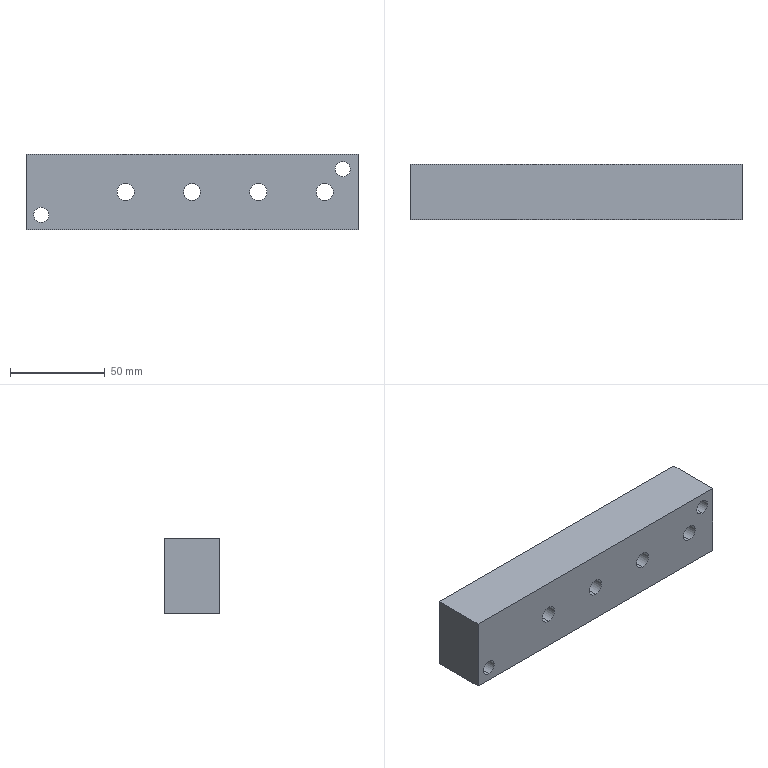Component | SolidWorks | Box151BackingPlateDowelPin-1 | 1 solid | 33 faces | box 175 x 29 x 40 mm | volume 185555 mm3 | cylinder 22 | plane 11 | commonest cylinder face diameters 15 x8 9 x8 8 x4 14 x2
build123d program:
from build123d import *

# Parameters (mm, degrees)
SKETCH1_W                                       = 175
SKETCH1_H                                       = 40
BOSS_EXTRUDE1_DEPTH                             = 29
SKETCH2_R                                       = 7
CUT_EXTRUDE1_DEPTH                              = 20
M8_HEX_SOCKET_HEAD_CAP_SCREW_CBORE1_D           = 9
M8_HEX_SOCKET_HEAD_CAP_SCREW_CBORE1_CBORE_D     = 15
M8_HEX_SOCKET_HEAD_CAP_SCREW_CBORE1_CBORE_DEPTH = 9
SKETCH6_R                                       = 4
CUT_EXTRUDE2_DEPTH                              = 50


with BuildPart() as part:
    # Sketch1 → Boss-Extrude1 (new body)
    with BuildSketch(Plane(origin=(0, 0, 0), x_dir=(1, 0, 0), z_dir=(0, 1, 0))):
        Rectangle(SKETCH1_W, SKETCH1_H)
    extrude(amount=BOSS_EXTRUDE1_DEPTH)

    # Sketch2 → Cut-Extrude1 (cut)
    with BuildSketch(Plane(origin=(0, 29, 0), x_dir=(1, 0, 0), z_dir=(0, 1, 0))):
        with Locations(Location((-67, 2, 0), (0, 0, 270))):
            Circle(SKETCH2_R)
    extrude(amount=-CUT_EXTRUDE1_DEPTH, mode=Mode.SUBTRACT)

    # M8 Hex Socket Head Cap Screw CBORE1 (through all)
    with Locations(Plane(origin=(0, 29, 0), x_dir=(1, 0, 0), z_dir=(0, 1, 0))):
        with Locations((-35, 0), (0, 0), (35, 0), (70, 0)):
            CounterBoreHole(M8_HEX_SOCKET_HEAD_CAP_SCREW_CBORE1_D / 2, M8_HEX_SOCKET_HEAD_CAP_SCREW_CBORE1_CBORE_D / 2, M8_HEX_SOCKET_HEAD_CAP_SCREW_CBORE1_CBORE_DEPTH)

    # Sketch6 → Cut-Extrude2 (cut)
    with BuildSketch(Plane(origin=(0, 29, 0), x_dir=(1, 0, 0), z_dir=(0, 1, 0))):
        with Locations(Location((-79.5, 12, 0), (0, 0, 270))):
            Circle(SKETCH6_R)
        with Locations(Location((79.5, -12, 0), (0, 0, 270))):
            Circle(SKETCH6_R)
    extrude(amount=-CUT_EXTRUDE2_DEPTH, mode=Mode.SUBTRACT)


solid = part.part

# Placed as in the assembly
solid = solid.moved(Location((-3.619, 64.047, -50), (0, 0, 0)))
STEP:
#1=CARTESIAN_POINT('',(-3.272,2.522,-2.283));
#2=VERTEX_POINT('',#1);
#3=CARTESIAN_POINT('',(-3.272,2.522,-2.598));
#4=VERTEX_POINT('',#3);
#5=CARTESIAN_POINT('',(-3.272,2.522,-2.441));
#6=DIRECTION('',(0.,-1.,0.));
#7=DIRECTION('',(0.,0.,-1.));
#8=AXIS2_PLACEMENT_3D('',#5,#6,#7);
#9=CIRCLE('',#8,0.1575);
#10=EDGE_CURVE('',#2,#4,#9,.T.);
#11=ORIENTED_EDGE('',*,*,#10,.T.);
#12=CARTESIAN_POINT('',(-3.272,3.663,-2.598));
#13=VERTEX_POINT('',#12);
#14=CARTESIAN_POINT('',(-3.272,1.695,-2.598));
#15=DIRECTION('',(0.,1.,0.));
#16=VECTOR('',#15,39.37);
#17=LINE('',#14,#16);
#18=EDGE_CURVE('',#4,#13,#17,.T.);
#19=ORIENTED_EDGE('',*,*,#18,.T.);
#20=CARTESIAN_POINT('',(-3.272,3.663,-2.283));
#21=VERTEX_POINT('',#20);
#22=CARTESIAN_POINT('',(-3.272,3.663,-2.441));
#23=DIRECTION('',(0.,1.,0.));
#24=DIRECTION('',(0.,0.,1.));
#25=AXIS2_PLACEMENT_3D('',#22,#23,#24);
#26=CIRCLE('',#25,0.1575);
#27=EDGE_CURVE('',#13,#21,#26,.T.);
#28=ORIENTED_EDGE('',*,*,#27,.T.);
#29=CARTESIAN_POINT('',(-3.272,1.695,-2.283));
#30=DIRECTION('',(0.,1.,0.));
#31=VECTOR('',#30,39.37);
#32=LINE('',#29,#31);
#33=EDGE_CURVE('',#2,#21,#32,.T.);
#34=ORIENTED_EDGE('',*,*,#33,.F.);
#35=EDGE_LOOP('',(#11,#19,#28,#34));
#36=FACE_OUTER_BOUND('',#35,.T.);
#37=CARTESIAN_POINT('',(-3.272,1.695,-2.441));
#38=DIRECTION('',(0.,1.,0.));
#39=DIRECTION('',(0.,0.,1.));
#40=AXIS2_PLACEMENT_3D('',#37,#38,#39);
#41=CYLINDRICAL_SURFACE('',#40,0.1575);
#42=ADVANCED_FACE('',(#36),#41,.F.);
#43=CARTESIAN_POINT('',(2.987,2.522,-1.339));
#44=VERTEX_POINT('',#43);
#45=CARTESIAN_POINT('',(2.987,2.522,-1.654));
#46=VERTEX_POINT('',#45);
#47=CARTESIAN_POINT('',(2.987,2.522,-1.496));
#48=DIRECTION('',(0.,-1.,0.));
#49=DIRECTION('',(0.,0.,-1.));
#50=AXIS2_PLACEMENT_3D('',#47,#48,#49);
#51=CIRCLE('',#50,0.1575);
#52=EDGE_CURVE('',#44,#46,#51,.T.);
#53=ORIENTED_EDGE('',*,*,#52,.T.);
#54=CARTESIAN_POINT('',(2.987,3.663,-1.654));
#55=VERTEX_POINT('',#54);
#56=CARTESIAN_POINT('',(2.987,1.695,-1.654));
#57=DIRECTION('',(0.,1.,0.));
#58=VECTOR('',#57,39.37);
#59=LINE('',#56,#58);
#60=EDGE_CURVE('',#46,#55,#59,.T.);
#61=ORIENTED_EDGE('',*,*,#60,.T.);
#62=CARTESIAN_POINT('',(2.987,3.663,-1.339));
#63=VERTEX_POINT('',#62);
#64=CARTESIAN_POINT('',(2.987,3.663,-1.496));
#65=DIRECTION('',(0.,1.,0.));
#66=DIRECTION('',(0.,0.,1.));
#67=AXIS2_PLACEMENT_3D('',#64,#65,#66);
#68=CIRCLE('',#67,0.1575);
#69=EDGE_CURVE('',#55,#63,#68,.T.);
#70=ORIENTED_EDGE('',*,*,#69,.T.);
#71=CARTESIAN_POINT('',(2.987,1.695,-1.339));
#72=DIRECTION('',(0.,1.,0.));
#73=VECTOR('',#72,39.37);
#74=LINE('',#71,#73);
#75=EDGE_CURVE('',#44,#63,#74,.T.);
#76=ORIENTED_EDGE('',*,*,#75,.F.);
#77=EDGE_LOOP('',(#53,#61,#70,#76));
#78=FACE_OUTER_BOUND('',#77,.T.);
#79=CARTESIAN_POINT('',(2.987,1.695,-1.496));
#80=DIRECTION('',(0.,1.,0.));
#81=DIRECTION('',(0.,0.,1.));
#82=AXIS2_PLACEMENT_3D('',#79,#80,#81);
#83=CYLINDRICAL_SURFACE('',#82,0.1575);
#84=ADVANCED_FACE('',(#78),#83,.F.);
#85=CARTESIAN_POINT('',(-1.52,3.309,-2.264));
#86=VERTEX_POINT('',#85);
#87=CARTESIAN_POINT('',(-1.52,3.309,-1.673));
#88=VERTEX_POINT('',#87);
#89=CARTESIAN_POINT('',(-1.52,3.309,-1.969));
#90=DIRECTION('',(0.,1.,0.));
#91=DIRECTION('',(0.,0.,1.));
#92=AXIS2_PLACEMENT_3D('',#89,#90,#91);
#93=CIRCLE('',#92,0.2953);
#94=EDGE_CURVE('',#86,#88,#93,.T.);
#95=ORIENTED_EDGE('',*,*,#94,.F.);
#96=CARTESIAN_POINT('',(-1.52,3.663,-2.264));
#97=VERTEX_POINT('',#96);
#98=CARTESIAN_POINT('',(-1.52,3.663,-2.264));
#99=DIRECTION('',(0.,1.,0.));
#100=VECTOR('',#99,39.37);
#101=LINE('',#98,#100);
#102=EDGE_CURVE('',#86,#97,#101,.T.);
#103=ORIENTED_EDGE('',*,*,#102,.T.);
#104=CARTESIAN_POINT('',(-1.52,3.663,-1.673));
#105=VERTEX_POINT('',#104);
#106=CARTESIAN_POINT('',(-1.52,3.663,-1.969));
#107=DIRECTION('',(0.,1.,0.));
#108=DIRECTION('',(0.,0.,1.));
#109=AXIS2_PLACEMENT_3D('',#106,#107,#108);
#110=CIRCLE('',#109,0.2953);
#111=EDGE_CURVE('',#97,#105,#110,.T.);
#112=ORIENTED_EDGE('',*,*,#111,.T.);
#113=CARTESIAN_POINT('',(-1.52,3.663,-1.673));
#114=DIRECTION('',(0.,1.,0.));
#115=VECTOR('',#114,39.37);
#116=LINE('',#113,#115);
#117=EDGE_CURVE('',#88,#105,#116,.T.);
#118=ORIENTED_EDGE('',*,*,#117,.F.);
#119=EDGE_LOOP('',(#95,#103,#112,#118));
#120=FACE_OUTER_BOUND('',#119,.T.);
#121=CARTESIAN_POINT('',(-1.52,3.663,-1.969));
#122=DIRECTION('',(0.,1.,0.));
#123=DIRECTION('',(0.,0.,1.));
#124=AXIS2_PLACEMENT_3D('',#121,#122,#123);
#125=CYLINDRICAL_SURFACE('',#124,0.2953);
#126=ADVANCED_FACE('',(#120),#125,.F.);
#127=CARTESIAN_POINT('',(-1.52,2.522,-1.791));
#128=VERTEX_POINT('',#127);
#129=CARTESIAN_POINT('',(-1.52,2.522,-2.146));
#130=VERTEX_POINT('',#129);
#131=CARTESIAN_POINT('',(-1.52,2.522,-1.969));
#132=DIRECTION('',(0.,-1.,0.));
#133=DIRECTION('',(0.,0.,-1.));
#134=AXIS2_PLACEMENT_3D('',#131,#132,#133);
#135=CIRCLE('',#134,0.1772);
#136=EDGE_CURVE('',#128,#130,#135,.T.);
#137=ORIENTED_EDGE('',*,*,#136,.T.);
#138=CARTESIAN_POINT('',(-1.52,3.309,-2.146));
#139=VERTEX_POINT('',#138);
#140=CARTESIAN_POINT('',(-1.52,3.663,-2.146));
#141=DIRECTION('',(0.,1.,0.));
#142=VECTOR('',#141,39.37);
#143=LINE('',#140,#142);
#144=EDGE_CURVE('',#130,#139,#143,.T.);
#145=ORIENTED_EDGE('',*,*,#144,.T.);
#146=CARTESIAN_POINT('',(-1.52,3.309,-1.791));
#147=VERTEX_POINT('',#146);
#148=CARTESIAN_POINT('',(-1.52,3.309,-1.969));
#149=DIRECTION('',(0.,1.,0.));
#150=DIRECTION('',(0.,0.,1.));
#151=AXIS2_PLACEMENT_3D('',#148,#149,#150);
#152=CIRCLE('',#151,0.1772);
#153=EDGE_CURVE('',#139,#147,#152,.T.);
#154=ORIENTED_EDGE('',*,*,#153,.T.);
#155=CARTESIAN_POINT('',(-1.52,3.663,-1.791));
#156=DIRECTION('',(0.,1.,0.));
#157=VECTOR('',#156,39.37);
#158=LINE('',#155,#157);
#159=EDGE_CURVE('',#128,#147,#158,.T.);
#160=ORIENTED_EDGE('',*,*,#159,.F.);
#161=EDGE_LOOP('',(#137,#145,#154,#160));
#162=FACE_OUTER_BOUND('',#161,.T.);
#163=CARTESIAN_POINT('',(-1.52,3.663,-1.969));
#164=DIRECTION('',(0.,1.,0.));
#165=DIRECTION('',(0.,0.,1.));
#166=AXIS2_PLACEMENT_3D('',#163,#164,#165);
#167=CYLINDRICAL_SURFACE('',#166,0.1772);
#168=ADVANCED_FACE('',(#162),#167,.F.);
#169=CARTESIAN_POINT('',(-0.1425,3.309,-2.264));
#170=VERTEX_POINT('',#169);
#171=CARTESIAN_POINT('',(-0.1425,3.309,-1.673));
#172=VERTEX_POINT('',#171);
#173=CARTESIAN_POINT('',(-0.1425,3.309,-1.969));
#174=DIRECTION('',(0.,1.,0.));
#175=DIRECTION('',(0.,0.,1.));
#176=AXIS2_PLACEMENT_3D('',#173,#174,#175);
#177=CIRCLE('',#176,0.2953);
#178=EDGE_CURVE('',#170,#172,#177,.T.);
#179=ORIENTED_EDGE('',*,*,#178,.F.);
#180=CARTESIAN_POINT('',(-0.1425,3.663,-2.264));
#181=VERTEX_POINT('',#180);
#182=CARTESIAN_POINT('',(-0.1425,3.663,-2.264));
#183=DIRECTION('',(0.,1.,0.));
#184=VECTOR('',#183,39.37);
#185=LINE('',#182,#184);
#186=EDGE_CURVE('',#170,#181,#185,.T.);
#187=ORIENTED_EDGE('',*,*,#186,.T.);
#188=CARTESIAN_POINT('',(-0.1425,3.663,-1.673));
#189=VERTEX_POINT('',#188);
#190=CARTESIAN_POINT('',(-0.1425,3.663,-1.969));
#191=DIRECTION('',(0.,1.,0.));
#192=DIRECTION('',(0.,0.,1.));
#193=AXIS2_PLACEMENT_3D('',#190,#191,#192);
#194=CIRCLE('',#193,0.2953);
#195=EDGE_CURVE('',#181,#189,#194,.T.);
#196=ORIENTED_EDGE('',*,*,#195,.T.);
#197=CARTESIAN_POINT('',(-0.1425,3.663,-1.673));
#198=DIRECTION('',(0.,1.,0.));
#199=VECTOR('',#198,39.37);
#200=LINE('',#197,#199);
#201=EDGE_CURVE('',#172,#189,#200,.T.);
#202=ORIENTED_EDGE('',*,*,#201,.F.);
#203=EDGE_LOOP('',(#179,#187,#196,#202));
#204=FACE_OUTER_BOUND('',#203,.T.);
#205=CARTESIAN_POINT('',(-0.1425,3.663,-1.969));
#206=DIRECTION('',(0.,1.,0.));
#207=DIRECTION('',(0.,0.,1.));
#208=AXIS2_PLACEMENT_3D('',#205,#206,#207);
#209=CYLINDRICAL_SURFACE('',#208,0.2953);
#210=ADVANCED_FACE('',(#204),#209,.F.);
#211=CARTESIAN_POINT('',(-0.1425,2.522,-1.791));
#212=VERTEX_POINT('',#211);
#213=CARTESIAN_POINT('',(-0.1425,2.522,-2.146));
#214=VERTEX_POINT('',#213);
#215=CARTESIAN_POINT('',(-0.1425,2.522,-1.969));
#216=DIRECTION('',(0.,-1.,0.));
#217=DIRECTION('',(0.,0.,-1.));
#218=AXIS2_PLACEMENT_3D('',#215,#216,#217);
#219=CIRCLE('',#218,0.1772);
#220=EDGE_CURVE('',#212,#214,#219,.T.);
#221=ORIENTED_EDGE('',*,*,#220,.T.);
#222=CARTESIAN_POINT('',(-0.1425,3.309,-2.146));
#223=VERTEX_POINT('',#222);
#224=CARTESIAN_POINT('',(-0.1425,3.663,-2.146));
#225=DIRECTION('',(0.,1.,0.));
#226=VECTOR('',#225,39.37);
#227=LINE('',#224,#226);
#228=EDGE_CURVE('',#214,#223,#227,.T.);
#229=ORIENTED_EDGE('',*,*,#228,.T.);
#230=CARTESIAN_POINT('',(-0.1425,3.309,-1.791));
#231=VERTEX_POINT('',#230);
#232=CARTESIAN_POINT('',(-0.1425,3.309,-1.969));
#233=DIRECTION('',(0.,1.,0.));
#234=DIRECTION('',(0.,0.,1.));
#235=AXIS2_PLACEMENT_3D('',#232,#233,#234);
#236=CIRCLE('',#235,0.1772);
#237=EDGE_CURVE('',#223,#231,#236,.T.);
#238=ORIENTED_EDGE('',*,*,#237,.T.);
#239=CARTESIAN_POINT('',(-0.1425,3.663,-1.791));
#240=DIRECTION('',(0.,1.,0.));
#241=VECTOR('',#240,39.37);
#242=LINE('',#239,#241);
#243=EDGE_CURVE('',#212,#231,#242,.T.);
#244=ORIENTED_EDGE('',*,*,#243,.F.);
#245=EDGE_LOOP('',(#221,#229,#238,#244));
#246=FACE_OUTER_BOUND('',#245,.T.);
#247=CARTESIAN_POINT('',(-0.1425,3.663,-1.969));
#248=DIRECTION('',(0.,1.,0.));
#249=DIRECTION('',(0.,0.,1.));
#250=AXIS2_PLACEMENT_3D('',#247,#248,#249);
#251=CYLINDRICAL_SURFACE('',#250,0.1772);
#252=ADVANCED_FACE('',(#246),#251,.F.);
#253=CARTESIAN_POINT('',(1.235,3.309,-2.264));
#254=VERTEX_POINT('',#253);
#255=CARTESIAN_POINT('',(1.235,3.309,-1.673));
#256=VERTEX_POINT('',#255);
#257=CARTESIAN_POINT('',(1.235,3.309,-1.969));
#258=DIRECTION('',(0.,1.,0.));
#259=DIRECTION('',(0.,0.,1.));
#260=AXIS2_PLACEMENT_3D('',#257,#258,#259);
#261=CIRCLE('',#260,0.2953);
#262=EDGE_CURVE('',#254,#256,#261,.T.);
#263=ORIENTED_EDGE('',*,*,#262,.F.);
#264=CARTESIAN_POINT('',(1.235,3.663,-2.264));
#265=VERTEX_POINT('',#264);
#266=CARTESIAN_POINT('',(1.235,3.663,-2.264));
#267=DIRECTION('',(0.,1.,0.));
#268=VECTOR('',#267,39.37);
#269=LINE('',#266,#268);
#270=EDGE_CURVE('',#254,#265,#269,.T.);
#271=ORIENTED_EDGE('',*,*,#270,.T.);
#272=CARTESIAN_POINT('',(1.235,3.663,-1.673));
#273=VERTEX_POINT('',#272);
#274=CARTESIAN_POINT('',(1.235,3.663,-1.969));
#275=DIRECTION('',(0.,1.,0.));
#276=DIRECTION('',(0.,0.,1.));
#277=AXIS2_PLACEMENT_3D('',#274,#275,#276);
#278=CIRCLE('',#277,0.2953);
#279=EDGE_CURVE('',#265,#273,#278,.T.);
#280=ORIENTED_EDGE('',*,*,#279,.T.);
#281=CARTESIAN_POINT('',(1.235,3.663,-1.673));
#282=DIRECTION('',(0.,1.,0.));
#283=VECTOR('',#282,39.37);
#284=LINE('',#281,#283);
#285=EDGE_CURVE('',#256,#273,#284,.T.);
#286=ORIENTED_EDGE('',*,*,#285,.F.);
#287=EDGE_LOOP('',(#263,#271,#280,#286));
#288=FACE_OUTER_BOUND('',#287,.T.);
#289=CARTESIAN_POINT('',(1.235,3.663,-1.969));
#290=DIRECTION('',(0.,1.,0.));
#291=DIRECTION('',(0.,0.,1.));
#292=AXIS2_PLACEMENT_3D('',#289,#290,#291);
#293=CYLINDRICAL_SURFACE('',#292,0.2953);
#294=ADVANCED_FACE('',(#288),#293,.F.);
#295=CARTESIAN_POINT('',(1.235,2.522,-1.791));
#296=VERTEX_POINT('',#295);
#297=CARTESIAN_POINT('',(1.235,2.522,-2.146));
#298=VERTEX_POINT('',#297);
#299=CARTESIAN_POINT('',(1.235,2.522,-1.969));
#300=DIRECTION('',(0.,-1.,0.));
#301=DIRECTION('',(0.,0.,-1.));
#302=AXIS2_PLACEMENT_3D('',#299,#300,#301);
#303=CIRCLE('',#302,0.1772);
#304=EDGE_CURVE('',#296,#298,#303,.T.);
#305=ORIENTED_EDGE('',*,*,#304,.T.);
#306=CARTESIAN_POINT('',(1.235,3.309,-2.146));
#307=VERTEX_POINT('',#306);
#308=CARTESIAN_POINT('',(1.235,3.663,-2.146));
#309=DIRECTION('',(0.,1.,0.));
#310=VECTOR('',#309,39.37);
#311=LINE('',#308,#310);
#312=EDGE_CURVE('',#298,#307,#311,.T.);
#313=ORIENTED_EDGE('',*,*,#312,.T.);
#314=CARTESIAN_POINT('',(1.235,3.309,-1.791));
#315=VERTEX_POINT('',#314);
#316=CARTESIAN_POINT('',(1.235,3.309,-1.969));
#317=DIRECTION('',(0.,1.,0.));
#318=DIRECTION('',(0.,0.,1.));
#319=AXIS2_PLACEMENT_3D('',#316,#317,#318);
#320=CIRCLE('',#319,0.1772);
#321=EDGE_CURVE('',#307,#315,#320,.T.);
#322=ORIENTED_EDGE('',*,*,#321,.T.);
#323=CARTESIAN_POINT('',(1.235,3.663,-1.791));
#324=DIRECTION('',(0.,1.,0.));
#325=VECTOR('',#324,39.37);
#326=LINE('',#323,#325);
#327=EDGE_CURVE('',#296,#315,#326,.T.);
#328=ORIENTED_EDGE('',*,*,#327,.F.);
#329=EDGE_LOOP('',(#305,#313,#322,#328));
#330=FACE_OUTER_BOUND('',#329,.T.);
#331=CARTESIAN_POINT('',(1.235,3.663,-1.969));
#332=DIRECTION('',(0.,1.,0.));
#333=DIRECTION('',(0.,0.,1.));
#334=AXIS2_PLACEMENT_3D('',#331,#332,#333);
#335=CYLINDRICAL_SURFACE('',#334,0.1772);
#336=ADVANCED_FACE('',(#330),#335,.F.);
#337=CARTESIAN_POINT('',(2.613,3.309,-2.264));
#338=VERTEX_POINT('',#337);
#339=CARTESIAN_POINT('',(2.613,3.309,-1.673));
#340=VERTEX_POINT('',#339);
#341=CARTESIAN_POINT('',(2.613,3.309,-1.969));
#342=DIRECTION('',(0.,1.,0.));
#343=DIRECTION('',(0.,0.,1.));
#344=AXIS2_PLACEMENT_3D('',#341,#342,#343);
#345=CIRCLE('',#344,0.2953);
#346=EDGE_CURVE('',#338,#340,#345,.T.);
#347=ORIENTED_EDGE('',*,*,#346,.F.);
#348=CARTESIAN_POINT('',(2.613,3.663,-2.264));
#349=VERTEX_POINT('',#348);
#350=CARTESIAN_POINT('',(2.613,3.663,-2.264));
#351=DIRECTION('',(0.,1.,0.));
#352=VECTOR('',#351,39.37);
#353=LINE('',#350,#352);
#354=EDGE_CURVE('',#338,#349,#353,.T.);
#355=ORIENTED_EDGE('',*,*,#354,.T.);
#356=CARTESIAN_POINT('',(2.613,3.663,-1.673));
#357=VERTEX_POINT('',#356);
#358=CARTESIAN_POINT('',(2.613,3.663,-1.969));
#359=DIRECTION('',(0.,1.,0.));
#360=DIRECTION('',(0.,0.,1.));
#361=AXIS2_PLACEMENT_3D('',#358,#359,#360);
#362=CIRCLE('',#361,0.2953);
#363=EDGE_CURVE('',#349,#357,#362,.T.);
#364=ORIENTED_EDGE('',*,*,#363,.T.);
#365=CARTESIAN_POINT('',(2.613,3.663,-1.673));
#366=DIRECTION('',(0.,1.,0.));
#367=VECTOR('',#366,39.37);
#368=LINE('',#365,#367);
#369=EDGE_CURVE('',#340,#357,#368,.T.);
#370=ORIENTED_EDGE('',*,*,#369,.F.);
#371=EDGE_LOOP('',(#347,#355,#364,#370));
#372=FACE_OUTER_BOUND('',#371,.T.);
#373=CARTESIAN_POINT('',(2.613,3.663,-1.969));
#374=DIRECTION('',(0.,1.,0.));
#375=DIRECTION('',(0.,0.,1.));
#376=AXIS2_PLACEMENT_3D('',#373,#374,#375);
#377=CYLINDRICAL_SURFACE('',#376,0.2953);
#378=ADVANCED_FACE('',(#372),#377,.F.);
#379=CARTESIAN_POINT('',(2.613,2.522,-1.791));
#380=VERTEX_POINT('',#379);
#381=CARTESIAN_POINT('',(2.613,2.522,-2.146));
#382=VERTEX_POINT('',#381);
#383=CARTESIAN_POINT('',(2.613,2.522,-1.969));
#384=DIRECTION('',(0.,-1.,0.));
#385=DIRECTION('',(0.,0.,-1.));
#386=AXIS2_PLACEMENT_3D('',#383,#384,#385);
#387=CIRCLE('',#386,0.1772);
#388=EDGE_CURVE('',#380,#382,#387,.T.);
#389=ORIENTED_EDGE('',*,*,#388,.T.);
#390=CARTESIAN_POINT('',(2.613,3.309,-2.146));
#391=VERTEX_POINT('',#390);
#392=CARTESIAN_POINT('',(2.613,3.663,-2.146));
#393=DIRECTION('',(0.,1.,0.));
#394=VECTOR('',#393,39.37);
#395=LINE('',#392,#394);
#396=EDGE_CURVE('',#382,#391,#395,.T.);
#397=ORIENTED_EDGE('',*,*,#396,.T.);
#398=CARTESIAN_POINT('',(2.613,3.309,-1.791));
#399=VERTEX_POINT('',#398);
#400=CARTESIAN_POINT('',(2.613,3.309,-1.969));
#401=DIRECTION('',(0.,1.,0.));
#402=DIRECTION('',(0.,0.,1.));
#403=AXIS2_PLACEMENT_3D('',#400,#401,#402);
#404=CIRCLE('',#403,0.1772);
#405=EDGE_CURVE('',#391,#399,#404,.T.);
#406=ORIENTED_EDGE('',*,*,#405,.T.);
#407=CARTESIAN_POINT('',(2.613,3.663,-1.791));
#408=DIRECTION('',(0.,1.,0.));
#409=VECTOR('',#408,39.37);
#410=LINE('',#407,#409);
#411=EDGE_CURVE('',#380,#399,#410,.T.);
#412=ORIENTED_EDGE('',*,*,#411,.F.);
#413=EDGE_LOOP('',(#389,#397,#406,#412));
#414=FACE_OUTER_BOUND('',#413,.T.);
#415=CARTESIAN_POINT('',(2.613,3.663,-1.969));
#416=DIRECTION('',(0.,1.,0.));
#417=DIRECTION('',(0.,0.,1.));
#418=AXIS2_PLACEMENT_3D('',#415,#416,#417);
#419=CYLINDRICAL_SURFACE('',#418,0.1772);
#420=ADVANCED_FACE('',(#414),#419,.F.);
#421=CARTESIAN_POINT('',(-2.78,2.876,-2.323));
#422=VERTEX_POINT('',#421);
#423=CARTESIAN_POINT('',(-2.78,2.876,-1.772));
#424=VERTEX_POINT('',#423);
#425=CARTESIAN_POINT('',(-2.78,2.876,-2.047));
#426=DIRECTION('',(0.,1.,0.));
#427=DIRECTION('',(0.,0.,1.));
#428=AXIS2_PLACEMENT_3D('',#425,#426,#427);
#429=CIRCLE('',#428,0.2756);
#430=EDGE_CURVE('',#422,#424,#429,.T.);
#431=ORIENTED_EDGE('',*,*,#430,.F.);
#432=CARTESIAN_POINT('',(-2.78,3.663,-2.323));
#433=VERTEX_POINT('',#432);
#434=CARTESIAN_POINT('',(-2.78,2.876,-2.323));
#435=DIRECTION('',(0.,1.,0.));
#436=VECTOR('',#435,39.37);
#437=LINE('',#434,#436);
#438=EDGE_CURVE('',#422,#433,#437,.T.);
#439=ORIENTED_EDGE('',*,*,#438,.T.);
#440=CARTESIAN_POINT('',(-2.78,3.663,-1.772));
#441=VERTEX_POINT('',#440);
#442=CARTESIAN_POINT('',(-2.78,3.663,-2.047));
#443=DIRECTION('',(0.,1.,0.));
#444=DIRECTION('',(0.,0.,1.));
#445=AXIS2_PLACEMENT_3D('',#442,#443,#444);
#446=CIRCLE('',#445,0.2756);
#447=EDGE_CURVE('',#433,#441,#446,.T.);
#448=ORIENTED_EDGE('',*,*,#447,.T.);
#449=CARTESIAN_POINT('',(-2.78,2.876,-1.772));
#450=DIRECTION('',(0.,1.,0.));
#451=VECTOR('',#450,39.37);
#452=LINE('',#449,#451);
#453=EDGE_CURVE('',#424,#441,#452,.T.);
#454=ORIENTED_EDGE('',*,*,#453,.F.);
#455=EDGE_LOOP('',(#431,#439,#448,#454));
#456=FACE_OUTER_BOUND('',#455,.T.);
#457=CARTESIAN_POINT('',(-2.78,2.876,-2.047));
#458=DIRECTION('',(0.,1.,0.));
#459=DIRECTION('',(0.,0.,1.));
#460=AXIS2_PLACEMENT_3D('',#457,#458,#459);
#461=CYLINDRICAL_SURFACE('',#460,0.2756);
#462=ADVANCED_FACE('',(#456),#461,.F.);
#463=CARTESIAN_POINT('',(3.302,2.522,-1.181));
#464=VERTEX_POINT('',#463);
#465=CARTESIAN_POINT('',(3.302,2.522,-2.756));
#466=VERTEX_POINT('',#465);
#467=CARTESIAN_POINT('',(3.302,2.522,-1.181));
#468=DIRECTION('',(0.,0.,-1.));
#469=VECTOR('',#468,39.37);
#470=LINE('',#467,#469);
#471=EDGE_CURVE('',#464,#466,#470,.T.);
#472=ORIENTED_EDGE('',*,*,#471,.T.);
#473=CARTESIAN_POINT('',(3.302,3.663,-2.756));
#474=VERTEX_POINT('',#473);
#475=CARTESIAN_POINT('',(3.302,3.663,-2.756));
#476=DIRECTION('',(0.,-1.,0.));
#477=VECTOR('',#476,39.37);
#478=LINE('',#475,#477);
#479=EDGE_CURVE('',#474,#466,#478,.T.);
#480=ORIENTED_EDGE('',*,*,#479,.F.);
#481=CARTESIAN_POINT('',(3.302,3.663,-1.181));
#482=VERTEX_POINT('',#481);
#483=CARTESIAN_POINT('',(3.302,3.663,-1.181));
#484=DIRECTION('',(0.,0.,-1.));
#485=VECTOR('',#484,39.37);
#486=LINE('',#483,#485);
#487=EDGE_CURVE('',#482,#474,#486,.T.);
#488=ORIENTED_EDGE('',*,*,#487,.F.);
#489=CARTESIAN_POINT('',(3.302,3.663,-1.181));
#490=DIRECTION('',(0.,-1.,0.));
#491=VECTOR('',#490,39.37);
#492=LINE('',#489,#491);
#493=EDGE_CURVE('',#482,#464,#492,.T.);
#494=ORIENTED_EDGE('',*,*,#493,.T.);
#495=EDGE_LOOP('',(#472,#480,#488,#494));
#496=FACE_OUTER_BOUND('',#495,.T.);
#497=CARTESIAN_POINT('',(3.302,3.663,-1.181));
#498=DIRECTION('',(-1.,0.,0.));
#499=DIRECTION('',(0.,0.,1.));
#500=AXIS2_PLACEMENT_3D('',#497,#498,#499);
#501=PLANE('',#500);
#502=ADVANCED_FACE('',(#496),#501,.F.);
#503=CARTESIAN_POINT('',(-3.587,2.522,-2.756));
#504=VERTEX_POINT('',#503);
#505=CARTESIAN_POINT('',(-3.587,2.522,-2.756));
#506=DIRECTION('',(-1.,0.,0.));
#507=VECTOR('',#506,39.37);
#508=LINE('',#505,#507);
#509=EDGE_CURVE('',#466,#504,#508,.T.);
#510=ORIENTED_EDGE('',*,*,#509,.T.);
#511=CARTESIAN_POINT('',(-3.587,3.663,-2.756));
#512=VERTEX_POINT('',#511);
#513=CARTESIAN_POINT('',(-3.587,3.663,-2.756));
#514=DIRECTION('',(0.,-1.,0.));
#515=VECTOR('',#514,39.37);
#516=LINE('',#513,#515);
#517=EDGE_CURVE('',#512,#504,#516,.T.);
#518=ORIENTED_EDGE('',*,*,#517,.F.);
#519=CARTESIAN_POINT('',(-3.587,3.663,-2.756));
#520=DIRECTION('',(-1.,0.,0.));
#521=VECTOR('',#520,39.37);
#522=LINE('',#519,#521);
#523=EDGE_CURVE('',#474,#512,#522,.T.);
#524=ORIENTED_EDGE('',*,*,#523,.F.);
#525=ORIENTED_EDGE('',*,*,#479,.T.);
#526=EDGE_LOOP('',(#510,#518,#524,#525));
#527=FACE_OUTER_BOUND('',#526,.T.);
#528=CARTESIAN_POINT('',(-3.587,3.663,-2.756));
#529=DIRECTION('',(0.,0.,1.));
#530=DIRECTION('',(1.,0.,0.));
#531=AXIS2_PLACEMENT_3D('',#528,#529,#530);
#532=PLANE('',#531);
#533=ADVANCED_FACE('',(#527),#532,.F.);
#534=CARTESIAN_POINT('',(-3.587,2.522,-1.181));
#535=VERTEX_POINT('',#534);
#536=CARTESIAN_POINT('',(-3.587,2.522,-1.181));
#537=DIRECTION('',(0.,0.,1.));
#538=VECTOR('',#537,39.37);
#539=LINE('',#536,#538);
#540=EDGE_CURVE('',#504,#535,#539,.T.);
#541=ORIENTED_EDGE('',*,*,#540,.T.);
#542=CARTESIAN_POINT('',(-3.587,3.663,-1.181));
#543=VERTEX_POINT('',#542);
#544=CARTESIAN_POINT('',(-3.587,3.663,-1.181));
#545=DIRECTION('',(0.,-1.,0.));
#546=VECTOR('',#545,39.37);
#547=LINE('',#544,#546);
#548=EDGE_CURVE('',#543,#535,#547,.T.);
#549=ORIENTED_EDGE('',*,*,#548,.F.);
#550=CARTESIAN_POINT('',(-3.587,3.663,-1.181));
#551=DIRECTION('',(0.,0.,1.));
#552=VECTOR('',#551,39.37);
#553=LINE('',#550,#552);
#554=EDGE_CURVE('',#512,#543,#553,.T.);
#555=ORIENTED_EDGE('',*,*,#554,.F.);
#556=ORIENTED_EDGE('',*,*,#517,.T.);
#557=EDGE_LOOP('',(#541,#549,#555,#556));
#558=FACE_OUTER_BOUND('',#557,.T.);
#559=CARTESIAN_POINT('',(-3.587,3.663,-1.181));
#560=DIRECTION('',(1.,0.,0.));
#561=DIRECTION('',(0.,0.,-1.));
#562=AXIS2_PLACEMENT_3D('',#559,#560,#561);
#563=PLANE('',#562);
#564=ADVANCED_FACE('',(#558),#563,.F.);
#565=CARTESIAN_POINT('',(-3.587,2.522,-1.181));
#566=DIRECTION('',(1.,0.,0.));
#567=VECTOR('',#566,39.37);
#568=LINE('',#565,#567);
#569=EDGE_CURVE('',#535,#464,#568,.T.);
#570=ORIENTED_EDGE('',*,*,#569,.T.);
#571=ORIENTED_EDGE('',*,*,#493,.F.);
#572=CARTESIAN_POINT('',(-3.587,3.663,-1.181));
#573=DIRECTION('',(1.,0.,0.));
#574=VECTOR('',#573,39.37);
#575=LINE('',#572,#574);
#576=EDGE_CURVE('',#543,#482,#575,.T.);
#577=ORIENTED_EDGE('',*,*,#576,.F.);
#578=ORIENTED_EDGE('',*,*,#548,.T.);
#579=EDGE_LOOP('',(#570,#571,#577,#578));
#580=FACE_OUTER_BOUND('',#579,.T.);
#581=CARTESIAN_POINT('',(-3.587,3.663,-1.181));
#582=DIRECTION('',(0.,0.,-1.));
#583=DIRECTION('',(-1.,0.,0.));
#584=AXIS2_PLACEMENT_3D('',#581,#582,#583);
#585=PLANE('',#584);
#586=ADVANCED_FACE('',(#580),#585,.F.);
#587=CARTESIAN_POINT('',(-3.272,3.663,-2.441));
#588=DIRECTION('',(0.,1.,0.));
#589=DIRECTION('',(0.,0.,1.));
#590=AXIS2_PLACEMENT_3D('',#587,#588,#589);
#591=CIRCLE('',#590,0.1575);
#592=EDGE_CURVE('',#21,#13,#591,.T.);
#593=ORIENTED_EDGE('',*,*,#592,.F.);
#594=ORIENTED_EDGE('',*,*,#27,.F.);
#595=EDGE_LOOP('',(#593,#594));
#596=FACE_BOUND('',#595,.T.);
#597=CARTESIAN_POINT('',(2.987,3.663,-1.496));
#598=DIRECTION('',(0.,1.,0.));
#599=DIRECTION('',(0.,0.,1.));
#600=AXIS2_PLACEMENT_3D('',#597,#598,#599);
#601=CIRCLE('',#600,0.1575);
#602=EDGE_CURVE('',#63,#55,#601,.T.);
#603=ORIENTED_EDGE('',*,*,#602,.F.);
#604=ORIENTED_EDGE('',*,*,#69,.F.);
#605=EDGE_LOOP('',(#603,#604));
#606=FACE_BOUND('',#605,.T.);
#607=CARTESIAN_POINT('',(-1.52,3.663,-1.969));
#608=DIRECTION('',(0.,1.,0.));
#609=DIRECTION('',(0.,0.,1.));
#610=AXIS2_PLACEMENT_3D('',#607,#608,#609);
#611=CIRCLE('',#610,0.2953);
#612=EDGE_CURVE('',#105,#97,#611,.T.);
#613=ORIENTED_EDGE('',*,*,#612,.F.);
#614=ORIENTED_EDGE('',*,*,#111,.F.);
#615=EDGE_LOOP('',(#613,#614));
#616=FACE_BOUND('',#615,.T.);
#617=CARTESIAN_POINT('',(-0.1425,3.663,-1.969));
#618=DIRECTION('',(0.,1.,0.));
#619=DIRECTION('',(0.,0.,1.));
#620=AXIS2_PLACEMENT_3D('',#617,#618,#619);
#621=CIRCLE('',#620,0.2953);
#622=EDGE_CURVE('',#189,#181,#621,.T.);
#623=ORIENTED_EDGE('',*,*,#622,.F.);
#624=ORIENTED_EDGE('',*,*,#195,.F.);
#625=EDGE_LOOP('',(#623,#624));
#626=FACE_BOUND('',#625,.T.);
#627=CARTESIAN_POINT('',(1.235,3.663,-1.969));
#628=DIRECTION('',(0.,1.,0.));
#629=DIRECTION('',(0.,0.,1.));
#630=AXIS2_PLACEMENT_3D('',#627,#628,#629);
#631=CIRCLE('',#630,0.2953);
#632=EDGE_CURVE('',#273,#265,#631,.T.);
#633=ORIENTED_EDGE('',*,*,#632,.F.);
#634=ORIENTED_EDGE('',*,*,#279,.F.);
#635=EDGE_LOOP('',(#633,#634));
#636=FACE_BOUND('',#635,.T.);
#637=CARTESIAN_POINT('',(2.613,3.663,-1.969));
#638=DIRECTION('',(0.,1.,0.));
#639=DIRECTION('',(0.,0.,1.));
#640=AXIS2_PLACEMENT_3D('',#637,#638,#639);
#641=CIRCLE('',#640,0.2953);
#642=EDGE_CURVE('',#357,#349,#641,.T.);
#643=ORIENTED_EDGE('',*,*,#642,.F.);
#644=ORIENTED_EDGE('',*,*,#363,.F.);
#645=EDGE_LOOP('',(#643,#644));
#646=FACE_BOUND('',#645,.T.);
#647=CARTESIAN_POINT('',(-2.78,3.663,-2.047));
#648=DIRECTION('',(0.,1.,0.));
#649=DIRECTION('',(0.,0.,1.));
#650=AXIS2_PLACEMENT_3D('',#647,#648,#649);
#651=CIRCLE('',#650,0.2756);
#652=EDGE_CURVE('',#441,#433,#651,.T.);
#653=ORIENTED_EDGE('',*,*,#652,.F.);
#654=ORIENTED_EDGE('',*,*,#447,.F.);
#655=EDGE_LOOP('',(#653,#654));
#656=FACE_BOUND('',#655,.T.);
#657=ORIENTED_EDGE('',*,*,#487,.T.);
#658=ORIENTED_EDGE('',*,*,#523,.T.);
#659=ORIENTED_EDGE('',*,*,#554,.T.);
#660=ORIENTED_EDGE('',*,*,#576,.T.);
#661=EDGE_LOOP('',(#657,#658,#659,#660));
#662=FACE_OUTER_BOUND('',#661,.T.);
#663=CARTESIAN_POINT('',(-0.1425,3.663,-1.969));
#664=DIRECTION('',(0.,-1.,0.));
#665=DIRECTION('',(0.,0.,-1.));
#666=AXIS2_PLACEMENT_3D('',#663,#664,#665);
#667=PLANE('',#666);
#668=ADVANCED_FACE('',(#596,#606,#616,#626,#636,#646,#656,#662),#667,.F.);
#669=ORIENTED_EDGE('',*,*,#10,.F.);
#670=CARTESIAN_POINT('',(-3.272,2.522,-2.441));
#671=DIRECTION('',(0.,-1.,0.));
#672=DIRECTION('',(0.,0.,-1.));
#673=AXIS2_PLACEMENT_3D('',#670,#671,#672);
#674=CIRCLE('',#673,0.1575);
#675=EDGE_CURVE('',#4,#2,#674,.T.);
#676=ORIENTED_EDGE('',*,*,#675,.F.);
#677=EDGE_LOOP('',(#669,#676));
#678=FACE_BOUND('',#677,.T.);
#679=ORIENTED_EDGE('',*,*,#52,.F.);
#680=CARTESIAN_POINT('',(2.987,2.522,-1.496));
#681=DIRECTION('',(0.,-1.,0.));
#682=DIRECTION('',(0.,0.,-1.));
#683=AXIS2_PLACEMENT_3D('',#680,#681,#682);
#684=CIRCLE('',#683,0.1575);
#685=EDGE_CURVE('',#46,#44,#684,.T.);
#686=ORIENTED_EDGE('',*,*,#685,.F.);
#687=EDGE_LOOP('',(#679,#686));
#688=FACE_BOUND('',#687,.T.);
#689=ORIENTED_EDGE('',*,*,#136,.F.);
#690=CARTESIAN_POINT('',(-1.52,2.522,-1.969));
#691=DIRECTION('',(0.,-1.,0.));
#692=DIRECTION('',(0.,0.,-1.));
#693=AXIS2_PLACEMENT_3D('',#690,#691,#692);
#694=CIRCLE('',#693,0.1772);
#695=EDGE_CURVE('',#130,#128,#694,.T.);
#696=ORIENTED_EDGE('',*,*,#695,.F.);
#697=EDGE_LOOP('',(#689,#696));
#698=FACE_BOUND('',#697,.T.);
#699=ORIENTED_EDGE('',*,*,#220,.F.);
#700=CARTESIAN_POINT('',(-0.1425,2.522,-1.969));
#701=DIRECTION('',(0.,-1.,0.));
#702=DIRECTION('',(0.,0.,-1.));
#703=AXIS2_PLACEMENT_3D('',#700,#701,#702);
#704=CIRCLE('',#703,0.1772);
#705=EDGE_CURVE('',#214,#212,#704,.T.);
#706=ORIENTED_EDGE('',*,*,#705,.F.);
#707=EDGE_LOOP('',(#699,#706));
#708=FACE_BOUND('',#707,.T.);
#709=ORIENTED_EDGE('',*,*,#304,.F.);
#710=CARTESIAN_POINT('',(1.235,2.522,-1.969));
#711=DIRECTION('',(0.,-1.,0.));
#712=DIRECTION('',(0.,0.,-1.));
#713=AXIS2_PLACEMENT_3D('',#710,#711,#712);
#714=CIRCLE('',#713,0.1772);
#715=EDGE_CURVE('',#298,#296,#714,.T.);
#716=ORIENTED_EDGE('',*,*,#715,.F.);
#717=EDGE_LOOP('',(#709,#716));
#718=FACE_BOUND('',#717,.T.);
#719=ORIENTED_EDGE('',*,*,#388,.F.);
#720=CARTESIAN_POINT('',(2.613,2.522,-1.969));
#721=DIRECTION('',(0.,-1.,0.));
#722=DIRECTION('',(0.,0.,-1.));
#723=AXIS2_PLACEMENT_3D('',#720,#721,#722);
#724=CIRCLE('',#723,0.1772);
#725=EDGE_CURVE('',#382,#380,#724,.T.);
#726=ORIENTED_EDGE('',*,*,#725,.F.);
#727=EDGE_LOOP('',(#719,#726));
#728=FACE_BOUND('',#727,.T.);
#729=ORIENTED_EDGE('',*,*,#471,.F.);
#730=ORIENTED_EDGE('',*,*,#569,.F.);
#731=ORIENTED_EDGE('',*,*,#540,.F.);
#732=ORIENTED_EDGE('',*,*,#509,.F.);
#733=EDGE_LOOP('',(#729,#730,#731,#732));
#734=FACE_OUTER_BOUND('',#733,.T.);
#735=CARTESIAN_POINT('',(-0.1425,2.522,-1.969));
#736=DIRECTION('',(0.,-1.,0.));
#737=DIRECTION('',(0.,0.,-1.));
#738=AXIS2_PLACEMENT_3D('',#735,#736,#737);
#739=PLANE('',#738);
#740=ADVANCED_FACE('',(#678,#688,#698,#708,#718,#728,#734),#739,.T.);
#741=ORIENTED_EDGE('',*,*,#438,.F.);
#742=CARTESIAN_POINT('',(-2.78,2.876,-2.047));
#743=DIRECTION('',(0.,1.,0.));
#744=DIRECTION('',(0.,0.,1.));
#745=AXIS2_PLACEMENT_3D('',#742,#743,#744);
#746=CIRCLE('',#745,0.2756);
#747=EDGE_CURVE('',#424,#422,#746,.T.);
#748=ORIENTED_EDGE('',*,*,#747,.F.);
#749=ORIENTED_EDGE('',*,*,#453,.T.);
#750=ORIENTED_EDGE('',*,*,#652,.T.);
#751=EDGE_LOOP('',(#741,#748,#749,#750));
#752=FACE_OUTER_BOUND('',#751,.T.);
#753=CARTESIAN_POINT('',(-2.78,2.876,-2.047));
#754=DIRECTION('',(0.,1.,0.));
#755=DIRECTION('',(0.,0.,1.));
#756=AXIS2_PLACEMENT_3D('',#753,#754,#755);
#757=CYLINDRICAL_SURFACE('',#756,0.2756);
#758=ADVANCED_FACE('',(#752),#757,.F.);
#759=ORIENTED_EDGE('',*,*,#747,.T.);
#760=ORIENTED_EDGE('',*,*,#430,.T.);
#761=EDGE_LOOP('',(#759,#760));
#762=FACE_OUTER_BOUND('',#761,.T.);
#763=CARTESIAN_POINT('',(-2.78,2.876,-2.047));
#764=DIRECTION('',(0.,1.,0.));
#765=DIRECTION('',(0.,0.,1.));
#766=AXIS2_PLACEMENT_3D('',#763,#764,#765);
#767=PLANE('',#766);
#768=ADVANCED_FACE('',(#762),#767,.T.);
#769=ORIENTED_EDGE('',*,*,#396,.F.);
#770=ORIENTED_EDGE('',*,*,#725,.T.);
#771=ORIENTED_EDGE('',*,*,#411,.T.);
#772=CARTESIAN_POINT('',(2.613,3.309,-1.969));
#773=DIRECTION('',(0.,1.,0.));
#774=DIRECTION('',(0.,0.,1.));
#775=AXIS2_PLACEMENT_3D('',#772,#773,#774);
#776=CIRCLE('',#775,0.1772);
#777=EDGE_CURVE('',#399,#391,#776,.T.);
#778=ORIENTED_EDGE('',*,*,#777,.T.);
#779=EDGE_LOOP('',(#769,#770,#771,#778));
#780=FACE_OUTER_BOUND('',#779,.T.);
#781=CARTESIAN_POINT('',(2.613,3.663,-1.969));
#782=DIRECTION('',(0.,1.,0.));
#783=DIRECTION('',(0.,0.,1.));
#784=AXIS2_PLACEMENT_3D('',#781,#782,#783);
#785=CYLINDRICAL_SURFACE('',#784,0.1772);
#786=ADVANCED_FACE('',(#780),#785,.F.);
#787=ORIENTED_EDGE('',*,*,#777,.F.);
#788=ORIENTED_EDGE('',*,*,#405,.F.);
#789=EDGE_LOOP('',(#787,#788));
#790=FACE_BOUND('',#789,.T.);
#791=CARTESIAN_POINT('',(2.613,3.309,-1.969));
#792=DIRECTION('',(0.,1.,0.));
#793=DIRECTION('',(0.,0.,1.));
#794=AXIS2_PLACEMENT_3D('',#791,#792,#793);
#795=CIRCLE('',#794,0.2953);
#796=EDGE_CURVE('',#340,#338,#795,.T.);
#797=ORIENTED_EDGE('',*,*,#796,.T.);
#798=ORIENTED_EDGE('',*,*,#346,.T.);
#799=EDGE_LOOP('',(#797,#798));
#800=FACE_OUTER_BOUND('',#799,.T.);
#801=CARTESIAN_POINT('',(2.791,3.309,-1.969));
#802=DIRECTION('',(0.,-1.,0.));
#803=DIRECTION('',(0.,0.,-1.));
#804=AXIS2_PLACEMENT_3D('',#801,#802,#803);
#805=PLANE('',#804);
#806=ADVANCED_FACE('',(#790,#800),#805,.F.);
#807=ORIENTED_EDGE('',*,*,#354,.F.);
#808=ORIENTED_EDGE('',*,*,#796,.F.);
#809=ORIENTED_EDGE('',*,*,#369,.T.);
#810=ORIENTED_EDGE('',*,*,#642,.T.);
#811=EDGE_LOOP('',(#807,#808,#809,#810));
#812=FACE_OUTER_BOUND('',#811,.T.);
#813=CARTESIAN_POINT('',(2.613,3.663,-1.969));
#814=DIRECTION('',(0.,1.,0.));
#815=DIRECTION('',(0.,0.,1.));
#816=AXIS2_PLACEMENT_3D('',#813,#814,#815);
#817=CYLINDRICAL_SURFACE('',#816,0.2953);
#818=ADVANCED_FACE('',(#812),#817,.F.);
#819=ORIENTED_EDGE('',*,*,#312,.F.);
#820=ORIENTED_EDGE('',*,*,#715,.T.);
#821=ORIENTED_EDGE('',*,*,#327,.T.);
#822=CARTESIAN_POINT('',(1.235,3.309,-1.969));
#823=DIRECTION('',(0.,1.,0.));
#824=DIRECTION('',(0.,0.,1.));
#825=AXIS2_PLACEMENT_3D('',#822,#823,#824);
#826=CIRCLE('',#825,0.1772);
#827=EDGE_CURVE('',#315,#307,#826,.T.);
#828=ORIENTED_EDGE('',*,*,#827,.T.);
#829=EDGE_LOOP('',(#819,#820,#821,#828));
#830=FACE_OUTER_BOUND('',#829,.T.);
#831=CARTESIAN_POINT('',(1.235,3.663,-1.969));
#832=DIRECTION('',(0.,1.,0.));
#833=DIRECTION('',(0.,0.,1.));
#834=AXIS2_PLACEMENT_3D('',#831,#832,#833);
#835=CYLINDRICAL_SURFACE('',#834,0.1772);
#836=ADVANCED_FACE('',(#830),#835,.F.);
#837=ORIENTED_EDGE('',*,*,#827,.F.);
#838=ORIENTED_EDGE('',*,*,#321,.F.);
#839=EDGE_LOOP('',(#837,#838));
#840=FACE_BOUND('',#839,.T.);
#841=CARTESIAN_POINT('',(1.235,3.309,-1.969));
#842=DIRECTION('',(0.,1.,0.));
#843=DIRECTION('',(0.,0.,1.));
#844=AXIS2_PLACEMENT_3D('',#841,#842,#843);
#845=CIRCLE('',#844,0.2953);
#846=EDGE_CURVE('',#256,#254,#845,.T.);
#847=ORIENTED_EDGE('',*,*,#846,.T.);
#848=ORIENTED_EDGE('',*,*,#262,.T.);
#849=EDGE_LOOP('',(#847,#848));
#850=FACE_OUTER_BOUND('',#849,.T.);
#851=CARTESIAN_POINT('',(1.413,3.309,-1.969));
#852=DIRECTION('',(0.,-1.,0.));
#853=DIRECTION('',(0.,0.,-1.));
#854=AXIS2_PLACEMENT_3D('',#851,#852,#853);
#855=PLANE('',#854);
#856=ADVANCED_FACE('',(#840,#850),#855,.F.);
#857=ORIENTED_EDGE('',*,*,#270,.F.);
#858=ORIENTED_EDGE('',*,*,#846,.F.);
#859=ORIENTED_EDGE('',*,*,#285,.T.);
#860=ORIENTED_EDGE('',*,*,#632,.T.);
#861=EDGE_LOOP('',(#857,#858,#859,#860));
#862=FACE_OUTER_BOUND('',#861,.T.);
#863=CARTESIAN_POINT('',(1.235,3.663,-1.969));
#864=DIRECTION('',(0.,1.,0.));
#865=DIRECTION('',(0.,0.,1.));
#866=AXIS2_PLACEMENT_3D('',#863,#864,#865);
#867=CYLINDRICAL_SURFACE('',#866,0.2953);
#868=ADVANCED_FACE('',(#862),#867,.F.);
#869=ORIENTED_EDGE('',*,*,#228,.F.);
#870=ORIENTED_EDGE('',*,*,#705,.T.);
#871=ORIENTED_EDGE('',*,*,#243,.T.);
#872=CARTESIAN_POINT('',(-0.1425,3.309,-1.969));
#873=DIRECTION('',(0.,1.,0.));
#874=DIRECTION('',(0.,0.,1.));
#875=AXIS2_PLACEMENT_3D('',#872,#873,#874);
#876=CIRCLE('',#875,0.1772);
#877=EDGE_CURVE('',#231,#223,#876,.T.);
#878=ORIENTED_EDGE('',*,*,#877,.T.);
#879=EDGE_LOOP('',(#869,#870,#871,#878));
#880=FACE_OUTER_BOUND('',#879,.T.);
#881=CARTESIAN_POINT('',(-0.1425,3.663,-1.969));
#882=DIRECTION('',(0.,1.,0.));
#883=DIRECTION('',(0.,0.,1.));
#884=AXIS2_PLACEMENT_3D('',#881,#882,#883);
#885=CYLINDRICAL_SURFACE('',#884,0.1772);
#886=ADVANCED_FACE('',(#880),#885,.F.);
#887=ORIENTED_EDGE('',*,*,#877,.F.);
#888=ORIENTED_EDGE('',*,*,#237,.F.);
#889=EDGE_LOOP('',(#887,#888));
#890=FACE_BOUND('',#889,.T.);
#891=CARTESIAN_POINT('',(-0.1425,3.309,-1.969));
#892=DIRECTION('',(0.,1.,0.));
#893=DIRECTION('',(0.,0.,1.));
#894=AXIS2_PLACEMENT_3D('',#891,#892,#893);
#895=CIRCLE('',#894,0.2953);
#896=EDGE_CURVE('',#172,#170,#895,.T.);
#897=ORIENTED_EDGE('',*,*,#896,.T.);
#898=ORIENTED_EDGE('',*,*,#178,.T.);
#899=EDGE_LOOP('',(#897,#898));
#900=FACE_OUTER_BOUND('',#899,.T.);
#901=CARTESIAN_POINT('',(0.0347,3.309,-1.969));
#902=DIRECTION('',(0.,-1.,0.));
#903=DIRECTION('',(0.,0.,-1.));
#904=AXIS2_PLACEMENT_3D('',#901,#902,#903);
#905=PLANE('',#904);
#906=ADVANCED_FACE('',(#890,#900),#905,.F.);
#907=ORIENTED_EDGE('',*,*,#186,.F.);
#908=ORIENTED_EDGE('',*,*,#896,.F.);
#909=ORIENTED_EDGE('',*,*,#201,.T.);
#910=ORIENTED_EDGE('',*,*,#622,.T.);
#911=EDGE_LOOP('',(#907,#908,#909,#910));
#912=FACE_OUTER_BOUND('',#911,.T.);
#913=CARTESIAN_POINT('',(-0.1425,3.663,-1.969));
#914=DIRECTION('',(0.,1.,0.));
#915=DIRECTION('',(0.,0.,1.));
#916=AXIS2_PLACEMENT_3D('',#913,#914,#915);
#917=CYLINDRICAL_SURFACE('',#916,0.2953);
#918=ADVANCED_FACE('',(#912),#917,.F.);
#919=ORIENTED_EDGE('',*,*,#144,.F.);
#920=ORIENTED_EDGE('',*,*,#695,.T.);
#921=ORIENTED_EDGE('',*,*,#159,.T.);
#922=CARTESIAN_POINT('',(-1.52,3.309,-1.969));
#923=DIRECTION('',(0.,1.,0.));
#924=DIRECTION('',(0.,0.,1.));
#925=AXIS2_PLACEMENT_3D('',#922,#923,#924);
#926=CIRCLE('',#925,0.1772);
#927=EDGE_CURVE('',#147,#139,#926,.T.);
#928=ORIENTED_EDGE('',*,*,#927,.T.);
#929=EDGE_LOOP('',(#919,#920,#921,#928));
#930=FACE_OUTER_BOUND('',#929,.T.);
#931=CARTESIAN_POINT('',(-1.52,3.663,-1.969));
#932=DIRECTION('',(0.,1.,0.));
#933=DIRECTION('',(0.,0.,1.));
#934=AXIS2_PLACEMENT_3D('',#931,#932,#933);
#935=CYLINDRICAL_SURFACE('',#934,0.1772);
#936=ADVANCED_FACE('',(#930),#935,.F.);
#937=ORIENTED_EDGE('',*,*,#927,.F.);
#938=ORIENTED_EDGE('',*,*,#153,.F.);
#939=EDGE_LOOP('',(#937,#938));
#940=FACE_BOUND('',#939,.T.);
#941=CARTESIAN_POINT('',(-1.52,3.309,-1.969));
#942=DIRECTION('',(0.,1.,0.));
#943=DIRECTION('',(0.,0.,1.));
#944=AXIS2_PLACEMENT_3D('',#941,#942,#943);
#945=CIRCLE('',#944,0.2953);
#946=EDGE_CURVE('',#88,#86,#945,.T.);
#947=ORIENTED_EDGE('',*,*,#946,.T.);
#948=ORIENTED_EDGE('',*,*,#94,.T.);
#949=EDGE_LOOP('',(#947,#948));
#950=FACE_OUTER_BOUND('',#949,.T.);
#951=CARTESIAN_POINT('',(-1.343,3.309,-1.969));
#952=DIRECTION('',(0.,-1.,0.));
#953=DIRECTION('',(0.,0.,-1.));
#954=AXIS2_PLACEMENT_3D('',#951,#952,#953);
#955=PLANE('',#954);
#956=ADVANCED_FACE('',(#940,#950),#955,.F.);
#957=ORIENTED_EDGE('',*,*,#102,.F.);
#958=ORIENTED_EDGE('',*,*,#946,.F.);
#959=ORIENTED_EDGE('',*,*,#117,.T.);
#960=ORIENTED_EDGE('',*,*,#612,.T.);
#961=EDGE_LOOP('',(#957,#958,#959,#960));
#962=FACE_OUTER_BOUND('',#961,.T.);
#963=CARTESIAN_POINT('',(-1.52,3.663,-1.969));
#964=DIRECTION('',(0.,1.,0.));
#965=DIRECTION('',(0.,0.,1.));
#966=AXIS2_PLACEMENT_3D('',#963,#964,#965);
#967=CYLINDRICAL_SURFACE('',#966,0.2953);
#968=ADVANCED_FACE('',(#962),#967,.F.);
#969=ORIENTED_EDGE('',*,*,#60,.F.);
#970=ORIENTED_EDGE('',*,*,#685,.T.);
#971=ORIENTED_EDGE('',*,*,#75,.T.);
#972=ORIENTED_EDGE('',*,*,#602,.T.);
#973=EDGE_LOOP('',(#969,#970,#971,#972));
#974=FACE_OUTER_BOUND('',#973,.T.);
#975=CARTESIAN_POINT('',(2.987,1.695,-1.496));
#976=DIRECTION('',(0.,1.,0.));
#977=DIRECTION('',(0.,0.,1.));
#978=AXIS2_PLACEMENT_3D('',#975,#976,#977);
#979=CYLINDRICAL_SURFACE('',#978,0.1575);
#980=ADVANCED_FACE('',(#974),#979,.F.);
#981=ORIENTED_EDGE('',*,*,#18,.F.);
#982=ORIENTED_EDGE('',*,*,#675,.T.);
#983=ORIENTED_EDGE('',*,*,#33,.T.);
#984=ORIENTED_EDGE('',*,*,#592,.T.);
#985=EDGE_LOOP('',(#981,#982,#983,#984));
#986=FACE_OUTER_BOUND('',#985,.T.);
#987=CARTESIAN_POINT('',(-3.272,1.695,-2.441));
#988=DIRECTION('',(0.,1.,0.));
#989=DIRECTION('',(0.,0.,1.));
#990=AXIS2_PLACEMENT_3D('',#987,#988,#989);
#991=CYLINDRICAL_SURFACE('',#990,0.1575);
#992=ADVANCED_FACE('',(#986),#991,.F.);
#993=CLOSED_SHELL('',(#42,#84,#126,#168,#210,#252,#294,#336,#378,#420,#462,#502,#533,#564,#586,#668,#740,#758,#768,#786,#806,#818,#836,#856,#868,#886,#906,#918,#936,#956,#968,#980,#992));
#994=MANIFOLD_SOLID_BREP('',#993);
#995=CARTESIAN_POINT('',(0.,0.,0.));
#996=DIRECTION('',(0.,0.,1.));
#997=DIRECTION('',(1.,0.,0.));
#998=AXIS2_PLACEMENT_3D('',#995,#996,#997);
#999=(LENGTH_UNIT()NAMED_UNIT(*)SI_UNIT($,.METRE.));
#1000=LENGTH_MEASURE_WITH_UNIT(LENGTH_MEASURE(0.0254),#999);
#1001=DIMENSIONAL_EXPONENTS(1.,0.,0.,0.,0.,0.,0.);
#1002=(CONVERSION_BASED_UNIT('',#1000)LENGTH_UNIT()NAMED_UNIT(#1001));
#1003=UNCERTAINTY_MEASURE_WITH_UNIT(LENGTH_MEASURE(0.00001),#1002,'','');
#1004=(NAMED_UNIT(*)PLANE_ANGLE_UNIT()SI_UNIT($,.RADIAN.));
#1005=(NAMED_UNIT(*)SI_UNIT($,.STERADIAN.)SOLID_ANGLE_UNIT());
#1006=(GEOMETRIC_REPRESENTATION_CONTEXT(3)GLOBAL_UNCERTAINTY_ASSIGNED_CONTEXT((#1003))GLOBAL_UNIT_ASSIGNED_CONTEXT((#1002,#1004,#1005))REPRESENTATION_CONTEXT('',''));
#1007=ADVANCED_BREP_SHAPE_REPRESENTATION('',(#994,#998),#1006);
#1008=COLOUR_RGB('',0.7922,0.8196,0.9333);
#1009=FILL_AREA_STYLE_COLOUR('',#1008);
#1010=FILL_AREA_STYLE('',(#1009));
#1011=SURFACE_STYLE_FILL_AREA(#1010);
#1012=SURFACE_SIDE_STYLE('',(#1011));
#1013=SURFACE_STYLE_USAGE(.BOTH.,#1012);
#1014=PRESENTATION_STYLE_ASSIGNMENT((#1013));
#1015=STYLED_ITEM('',(#1014),#994);
#1016=(LENGTH_UNIT()NAMED_UNIT(*)SI_UNIT($,.METRE.));
#1017=LENGTH_MEASURE_WITH_UNIT(LENGTH_MEASURE(0.0254),#1016);
#1018=DIMENSIONAL_EXPONENTS(1.,0.,0.,0.,0.,0.,0.);
#1019=(CONVERSION_BASED_UNIT('',#1017)LENGTH_UNIT()NAMED_UNIT(#1018));
#1020=UNCERTAINTY_MEASURE_WITH_UNIT(LENGTH_MEASURE(0.00001),#1019,'','');
#1021=(NAMED_UNIT(*)PLANE_ANGLE_UNIT()SI_UNIT($,.RADIAN.));
#1022=(NAMED_UNIT(*)SI_UNIT($,.STERADIAN.)SOLID_ANGLE_UNIT());
#1023=(GEOMETRIC_REPRESENTATION_CONTEXT(3)GLOBAL_UNCERTAINTY_ASSIGNED_CONTEXT((#1020))GLOBAL_UNIT_ASSIGNED_CONTEXT((#1019,#1021,#1022))REPRESENTATION_CONTEXT('',''));
#1024=MECHANICAL_DESIGN_GEOMETRIC_PRESENTATION_REPRESENTATION('',(#1015),#1023);
#1025=PRESENTATION_LAYER_ASSIGNMENT('','',(#1015));